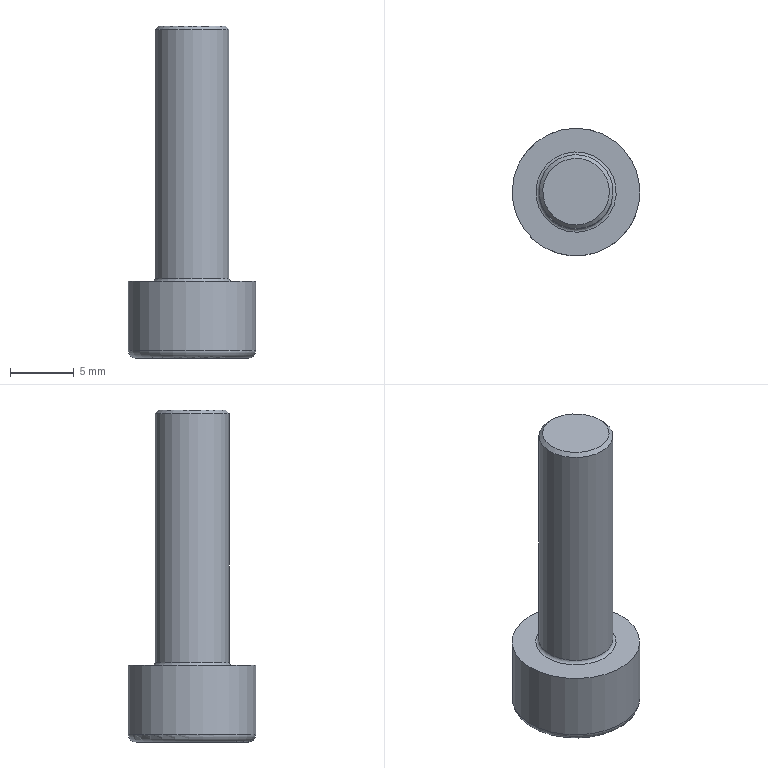Component | NX | GB-T70_1-2000_M6X20_2 | 1 solid | 27 faces | volume 906 mm3 | plane 15 | cone 8 | cylinder 2 | torus 2 | commonest cylinder face diameters 5.795 x1 10 x1